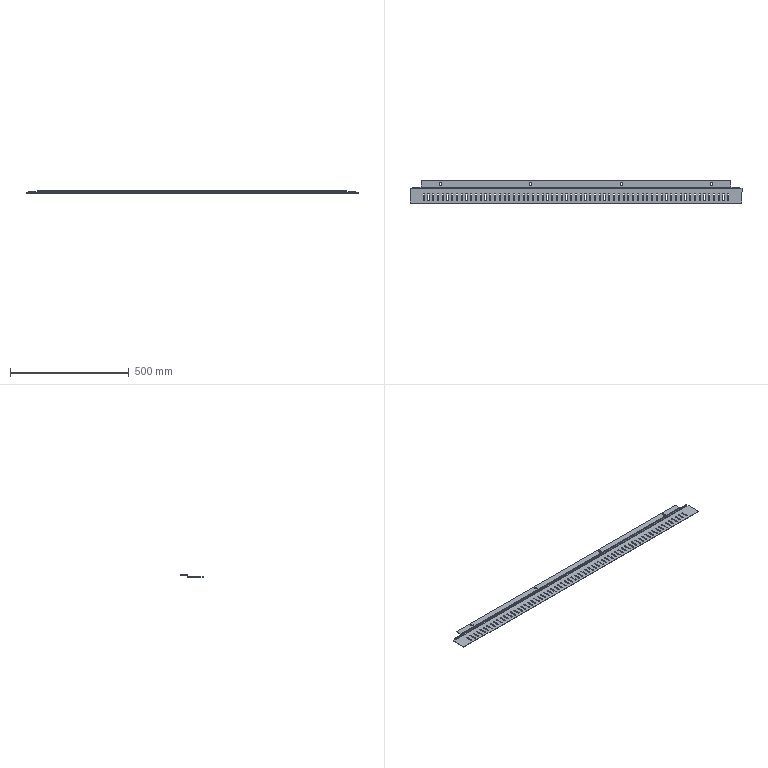Component | SolidWorks | TopCoverAssembly-1_TopCoverFrontAndRearFlange-3 | 1 solid | 369 faces | volume 190240 mm3 | cylinder 211 | plane 158 | commonest cylinder face diameters 5 x195 9 x12 6 x2 3 x2